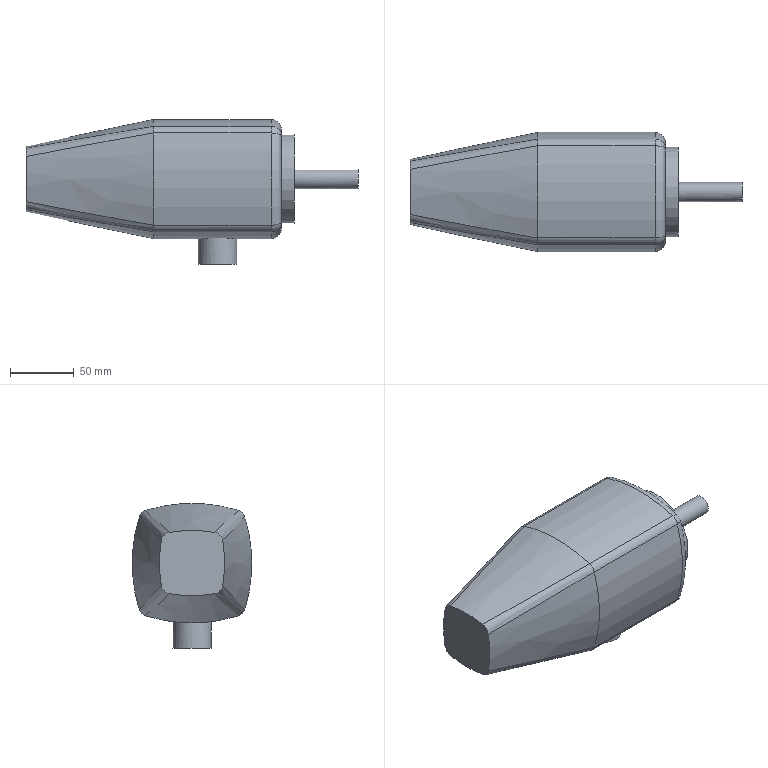Component | NX | MOTOR | 1 solid | 34 faces | volume 1325140 mm3 | cylinder 12 | plane 6 | cone 4 | spline 4 | sphere 4 | torus 4 | commonest cylinder face diameters 240 x4 16 x4 30 x1 25 x1 70 x1 15 x1